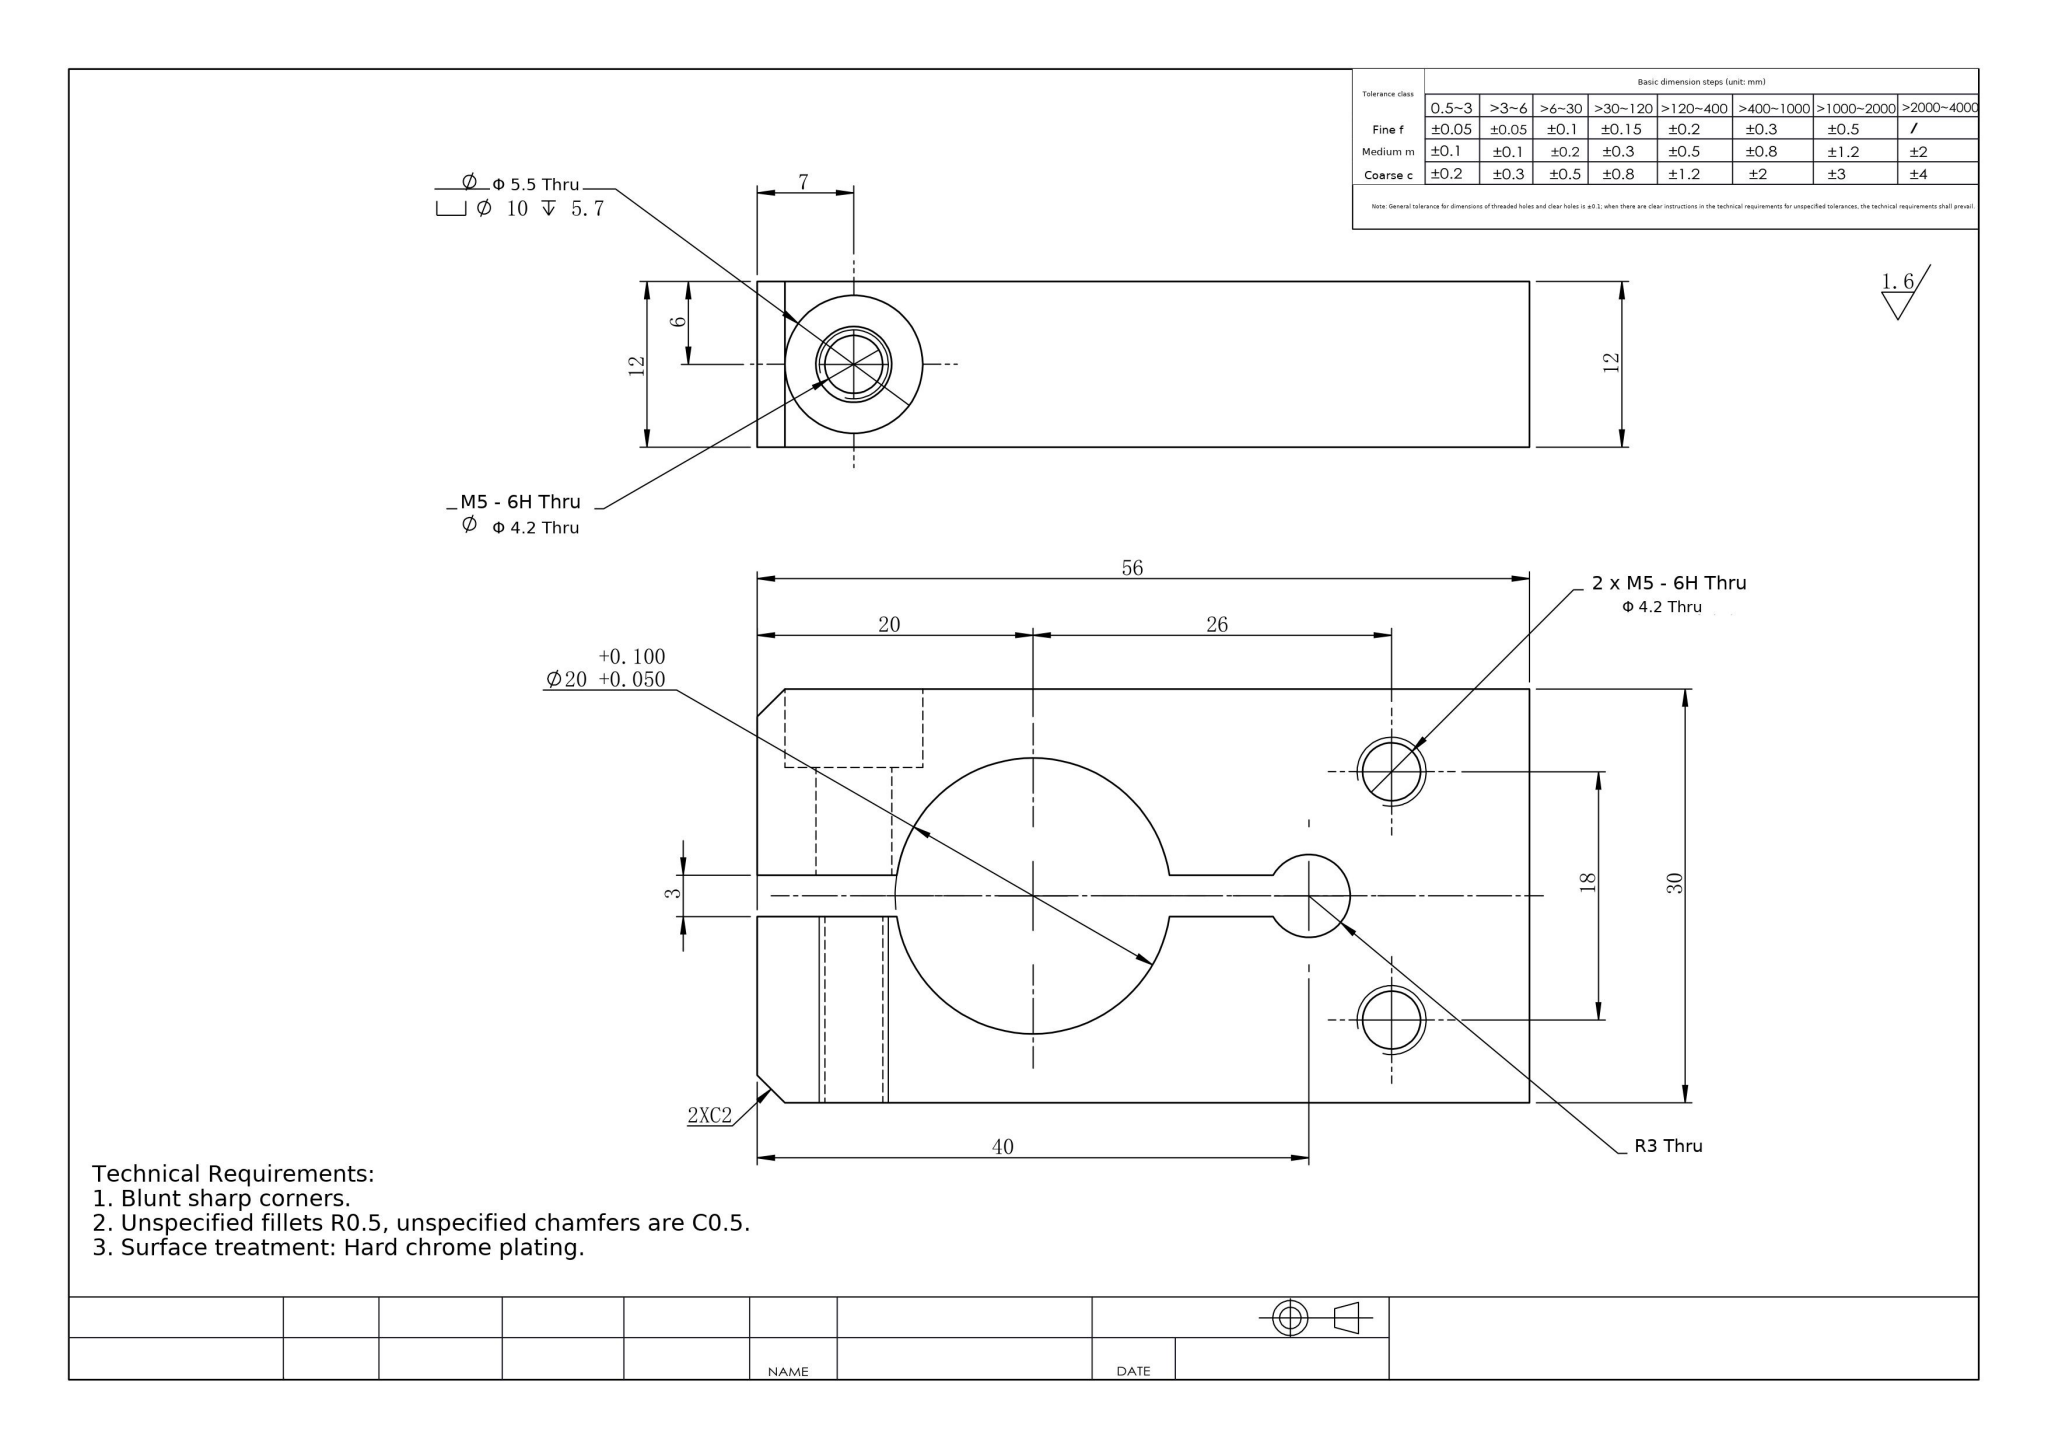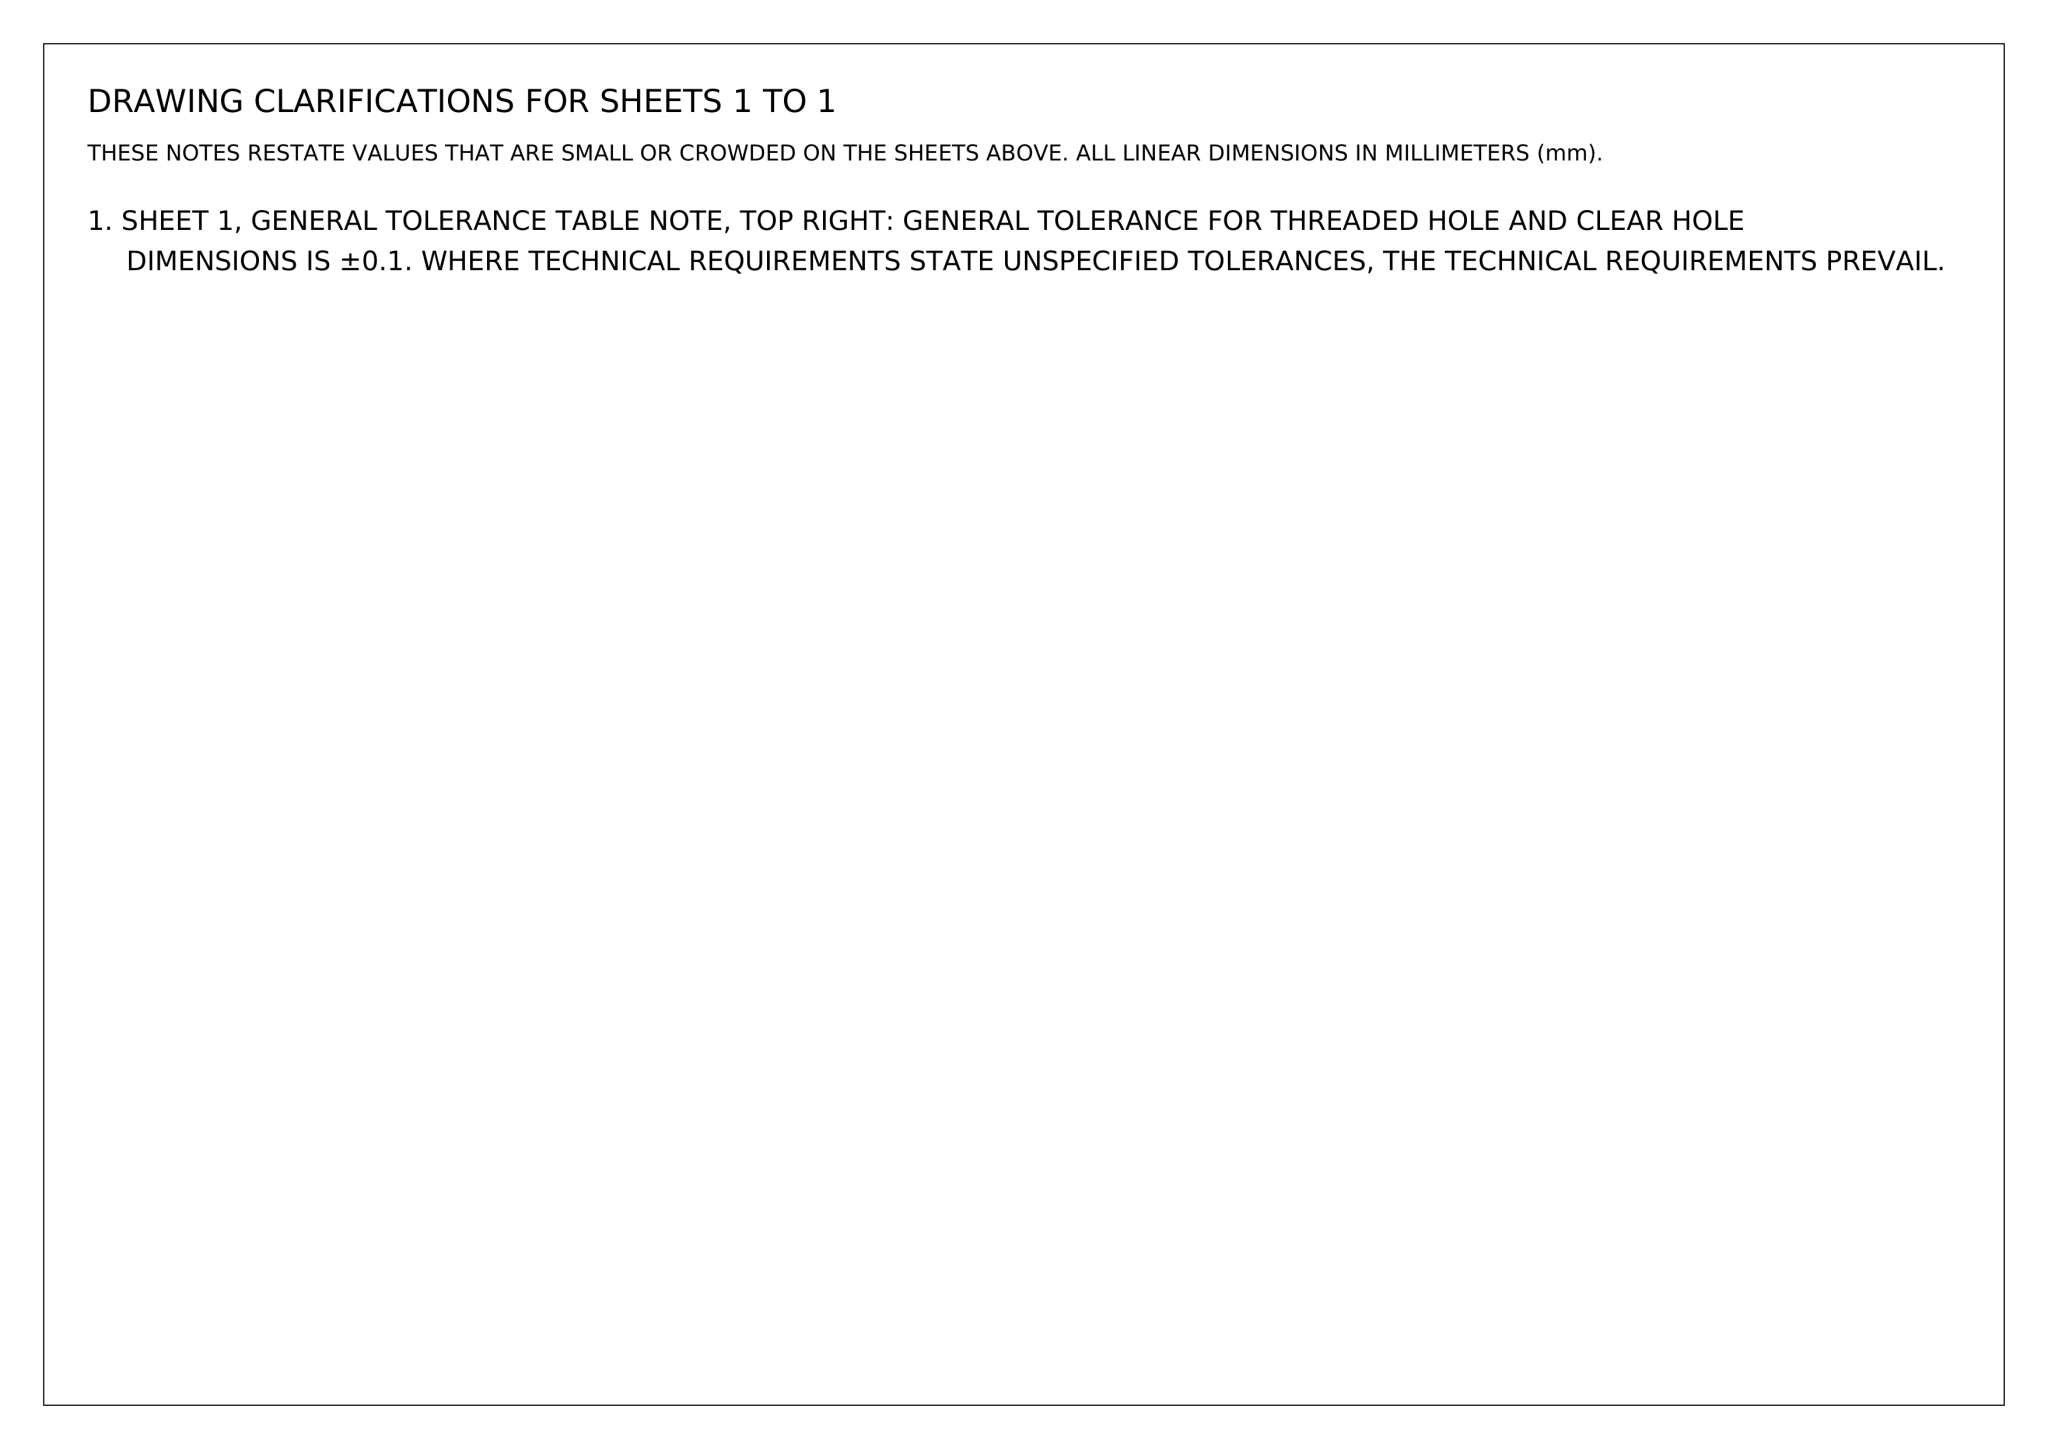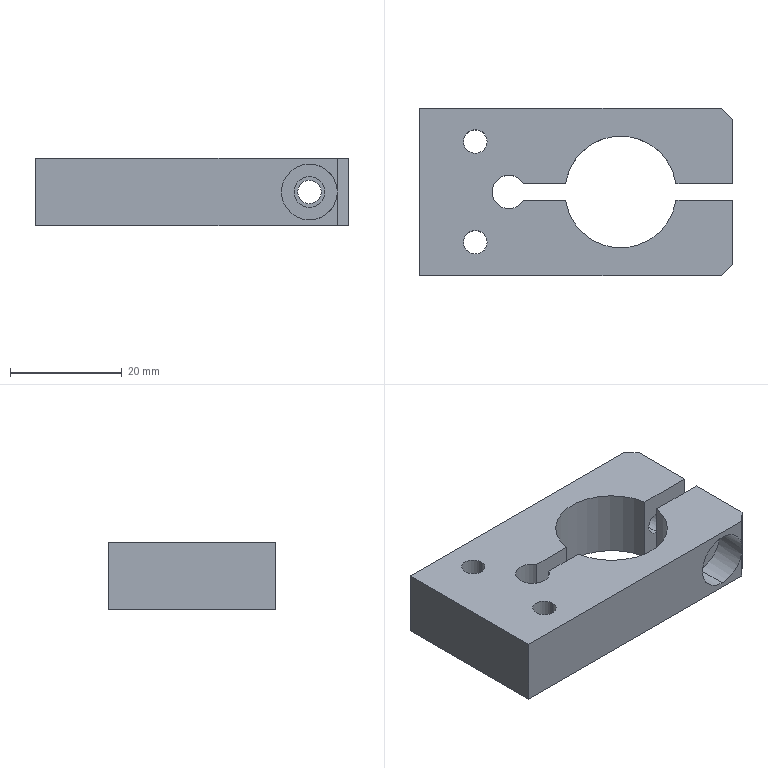Part | NX | mm | Stepped Cylindrical Cutout Mounting Block | 1 solid | 27 faces | box 56 x 30 x 12 mm | volume 14231 mm3 | plane 14 | cylinder 13 | commonest cylinder face diameters 4.2 x6 10 x2 5.5 x2 20 x2 6 x1